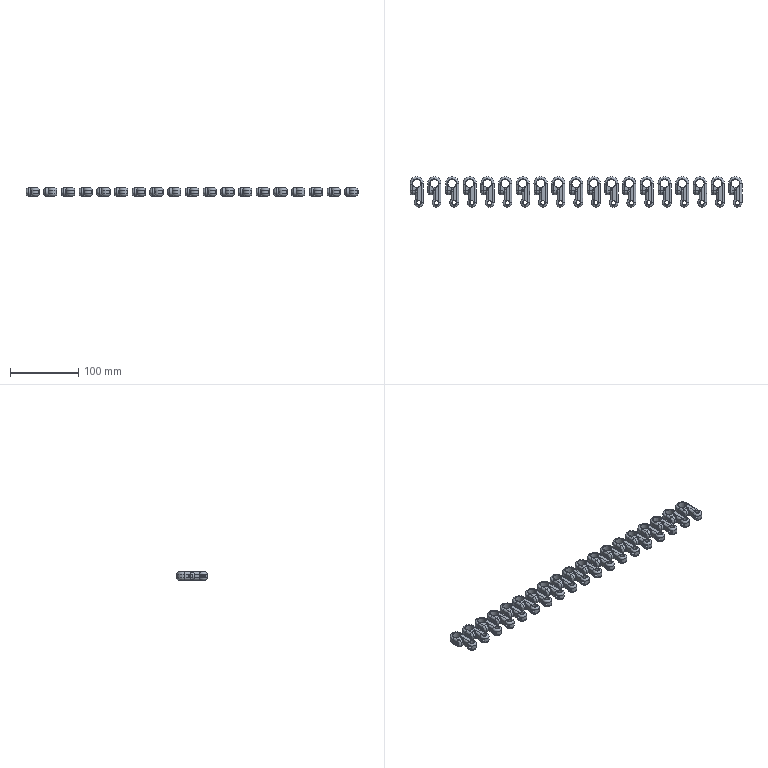CAM job | Mastercam | mm | 2 operations | part box 487.5 x 44.75 x 11.8
1. Contour (Ramp) | 9 - 8 平铣刀
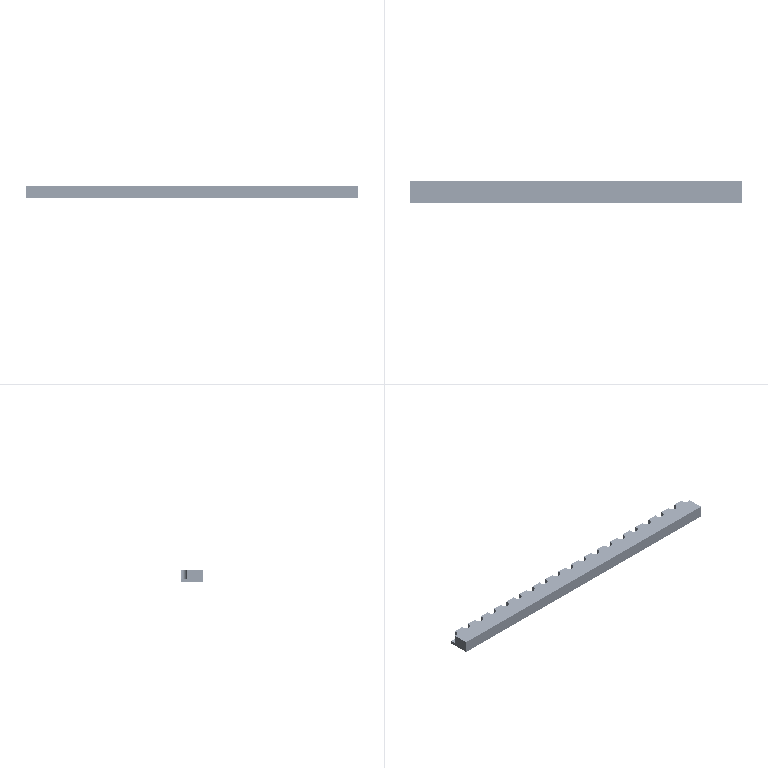2. Peck Drill | 5 - 6 钻头